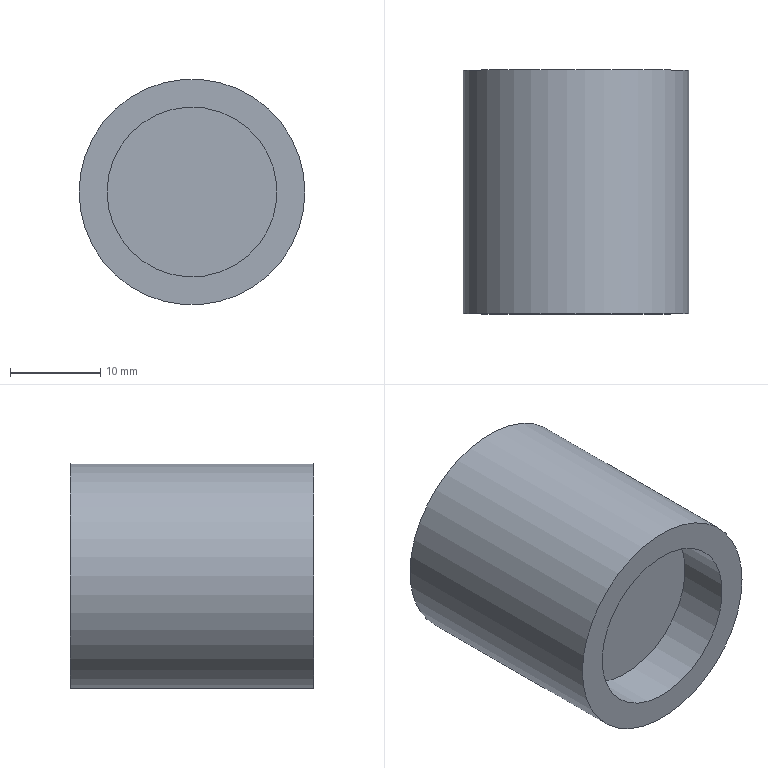Component | NX | SPRING_SEAT | 1 solid | 9 faces | box 25 x 27 x 25 mm | volume 9515 mm3 | plane 5 | cylinder 4 | commonest cylinder face diameters 10 x1 15.5 x1 25 x1 18.8 x1
STEP:
#1=CARTESIAN_POINT('',(0.,0.,0.));
#2=DIRECTION('',(0.,0.,1.));
#3=DIRECTION('',(1.,0.,0.));
#4=AXIS2_PLACEMENT_3D('',#1,#2,#3);
#5=CARTESIAN_POINT('',(38.195,58.009,0.));
#6=VERTEX_POINT('',#5);
#7=CARTESIAN_POINT('',(43.195,58.009,0.));
#8=DIRECTION('',(0.,1.,0.));
#9=DIRECTION('',(-1.,0.,0.));
#10=AXIS2_PLACEMENT_3D('',#7,#8,#9);
#11=CIRCLE('',#10,5.);
#12=CARTESIAN_POINT('',(38.195,58.009,0.));
#13=DIRECTION('',(-0.,-1.,0.));
#14=DIRECTION('',(1.,-0.,0.));
#15=AXIS2_PLACEMENT_3D('',#12,#13,#14);
#16=PLANE('',#15);
#17=CARTESIAN_POINT('',(0.,0.));
#18=CARTESIAN_POINT('',(0.,8.66));
#19=CARTESIAN_POINT('',(7.5,4.33));
#20=CARTESIAN_POINT('',(15.,0.));
#21=CARTESIAN_POINT('',(7.5,-4.33));
#22=CARTESIAN_POINT('',(0.,-8.66));
#23=CARTESIAN_POINT('',(0.,0.));
#24=(BOUNDED_CURVE()B_SPLINE_CURVE(2,(#17,#18,#19,#20,#21,#22,#23),.UNSPECIFIED.,.T.,.F.)B_SPLINE_CURVE_WITH_KNOTS((1,2,2,2,2,1),(-2.094,0.,2.094,4.189,6.283,8.378),.UNSPECIFIED.)CURVE()GEOMETRIC_REPRESENTATION_ITEM()RATIONAL_B_SPLINE_CURVE((1.,0.5,1.,0.5,1.,0.5,1.))REPRESENTATION_ITEM(''));
#25=(GEOMETRIC_REPRESENTATION_CONTEXT(2)PARAMETRIC_REPRESENTATION_CONTEXT()REPRESENTATION_CONTEXT('',''));
#26=DEFINITIONAL_REPRESENTATION('',(#24),#25);
#27=PCURVE('',#16,#26);
#28=CARTESIAN_POINT('',(43.195,78.009,0.));
#29=DIRECTION('',(0.,1.,0.));
#30=DIRECTION('',(-1.,0.,0.));
#31=AXIS2_PLACEMENT_3D('',#28,#29,#30);
#32=CYLINDRICAL_SURFACE('',#31,5.);
#33=CARTESIAN_POINT('',(0.,-20.));
#34=DIRECTION('',(1.,0.));
#35=VECTOR('',#34,1.);
#36=LINE('',#33,#35);
#37=(GEOMETRIC_REPRESENTATION_CONTEXT(2)PARAMETRIC_REPRESENTATION_CONTEXT()REPRESENTATION_CONTEXT('',''));
#38=DEFINITIONAL_REPRESENTATION('',(#36),#37);
#39=PCURVE('',#32,#38);
#40=SURFACE_CURVE('',#11,(#27,#39),.PCURVE_S1.);
#41=EDGE_CURVE('',#6,#6,#40,.T.);
#42=ORIENTED_EDGE('',*,*,#41,.T.);
#43=EDGE_LOOP('',(#42));
#44=FACE_BOUND('',#43,.T.);
#45=ADVANCED_FACE('',(#44),#16,.F.);
#46=ORIENTED_EDGE('',*,*,#41,.T.);
#47=CARTESIAN_POINT('',(38.195,67.809,0.));
#48=VERTEX_POINT('',#47);
#49=CARTESIAN_POINT('',(38.195,58.009,0.));
#50=CARTESIAN_POINT('',(38.195,67.809,0.));
#51=B_SPLINE_CURVE_WITH_KNOTS('',1,(#49,#50),.UNSPECIFIED.,.F.,.F.,(2,2),(-20.,-10.2),.PIECEWISE_BEZIER_KNOTS.);
#52=CARTESIAN_POINT('',(6.283,0.));
#53=DIRECTION('',(0.,1.));
#54=VECTOR('',#53,1.);
#55=LINE('',#52,#54);
#56=(GEOMETRIC_REPRESENTATION_CONTEXT(2)PARAMETRIC_REPRESENTATION_CONTEXT()REPRESENTATION_CONTEXT('',''));
#57=DEFINITIONAL_REPRESENTATION('',(#55),#56);
#58=PCURVE('',#32,#57);
#59=CARTESIAN_POINT('',(0.,0.));
#60=DIRECTION('',(0.,1.));
#61=VECTOR('',#60,1.);
#62=LINE('',#59,#61);
#63=(GEOMETRIC_REPRESENTATION_CONTEXT(2)PARAMETRIC_REPRESENTATION_CONTEXT()REPRESENTATION_CONTEXT('',''));
#64=DEFINITIONAL_REPRESENTATION('',(#62),#63);
#65=PCURVE('',#32,#64);
#66=SEAM_CURVE('',#51,(#58,#65),.PCURVE_S1.);
#67=EDGE_CURVE('',#6,#48,#66,.T.);
#68=ORIENTED_EDGE('',*,*,#67,.T.);
#69=CARTESIAN_POINT('',(43.195,67.809,0.));
#70=DIRECTION('',(0.,1.,0.));
#71=DIRECTION('',(-1.,0.,0.));
#72=AXIS2_PLACEMENT_3D('',#69,#70,#71);
#73=CIRCLE('',#72,5.);
#74=CARTESIAN_POINT('',(0.,-10.2));
#75=DIRECTION('',(1.,0.));
#76=VECTOR('',#75,1.);
#77=LINE('',#74,#76);
#78=(GEOMETRIC_REPRESENTATION_CONTEXT(2)PARAMETRIC_REPRESENTATION_CONTEXT()REPRESENTATION_CONTEXT('',''));
#79=DEFINITIONAL_REPRESENTATION('',(#77),#78);
#80=PCURVE('',#32,#79);
#81=CARTESIAN_POINT('',(35.445,67.809,0.));
#82=DIRECTION('',(-0.,-1.,0.));
#83=DIRECTION('',(1.,-0.,0.));
#84=AXIS2_PLACEMENT_3D('',#81,#82,#83);
#85=PLANE('',#84);
#86=CARTESIAN_POINT('',(2.75,0.));
#87=CARTESIAN_POINT('',(2.75,8.66));
#88=CARTESIAN_POINT('',(10.25,4.33));
#89=CARTESIAN_POINT('',(17.75,0.));
#90=CARTESIAN_POINT('',(10.25,-4.33));
#91=CARTESIAN_POINT('',(2.75,-8.66));
#92=CARTESIAN_POINT('',(2.75,0.));
#93=(BOUNDED_CURVE()B_SPLINE_CURVE(2,(#86,#87,#88,#89,#90,#91,#92),.UNSPECIFIED.,.T.,.F.)B_SPLINE_CURVE_WITH_KNOTS((1,2,2,2,2,1),(-2.094,0.,2.094,4.189,6.283,8.378),.UNSPECIFIED.)CURVE()GEOMETRIC_REPRESENTATION_ITEM()RATIONAL_B_SPLINE_CURVE((1.,0.5,1.,0.5,1.,0.5,1.))REPRESENTATION_ITEM(''));
#94=(GEOMETRIC_REPRESENTATION_CONTEXT(2)PARAMETRIC_REPRESENTATION_CONTEXT()REPRESENTATION_CONTEXT('',''));
#95=DEFINITIONAL_REPRESENTATION('',(#93),#94);
#96=PCURVE('',#85,#95);
#97=SURFACE_CURVE('',#73,(#80,#96),.PCURVE_S1.);
#98=EDGE_CURVE('',#48,#48,#97,.T.);
#99=ORIENTED_EDGE('',*,*,#98,.F.);
#100=ORIENTED_EDGE('',*,*,#67,.F.);
#101=EDGE_LOOP('',(#46,#68,#99,#100));
#102=FACE_BOUND('',#101,.F.);
#103=ADVANCED_FACE('',(#102),#32,.F.);
#104=ORIENTED_EDGE('',*,*,#98,.F.);
#105=EDGE_LOOP('',(#104));
#106=FACE_BOUND('',#105,.T.);
#107=CARTESIAN_POINT('',(35.445,67.809,0.));
#108=VERTEX_POINT('',#107);
#109=CARTESIAN_POINT('',(43.195,67.809,0.));
#110=DIRECTION('',(0.,1.,0.));
#111=DIRECTION('',(-1.,0.,0.));
#112=AXIS2_PLACEMENT_3D('',#109,#110,#111);
#113=CIRCLE('',#112,7.75);
#114=CARTESIAN_POINT('',(0.,0.));
#115=CARTESIAN_POINT('',(0.,13.423));
#116=CARTESIAN_POINT('',(11.625,6.712));
#117=CARTESIAN_POINT('',(23.25,0.));
#118=CARTESIAN_POINT('',(11.625,-6.712));
#119=CARTESIAN_POINT('',(0.,-13.423));
#120=CARTESIAN_POINT('',(0.,0.));
#121=(BOUNDED_CURVE()B_SPLINE_CURVE(2,(#114,#115,#116,#117,#118,#119,#120),.UNSPECIFIED.,.T.,.F.)B_SPLINE_CURVE_WITH_KNOTS((1,2,2,2,2,1),(-2.094,0.,2.094,4.189,6.283,8.378),.UNSPECIFIED.)CURVE()GEOMETRIC_REPRESENTATION_ITEM()RATIONAL_B_SPLINE_CURVE((1.,0.5,1.,0.5,1.,0.5,1.))REPRESENTATION_ITEM(''));
#122=(GEOMETRIC_REPRESENTATION_CONTEXT(2)PARAMETRIC_REPRESENTATION_CONTEXT()REPRESENTATION_CONTEXT('',''));
#123=DEFINITIONAL_REPRESENTATION('',(#121),#122);
#124=PCURVE('',#85,#123);
#125=CARTESIAN_POINT('',(43.195,78.009,0.));
#126=DIRECTION('',(0.,1.,0.));
#127=DIRECTION('',(-1.,0.,0.));
#128=AXIS2_PLACEMENT_3D('',#125,#126,#127);
#129=CYLINDRICAL_SURFACE('',#128,7.75);
#130=CARTESIAN_POINT('',(0.,-10.2));
#131=DIRECTION('',(1.,0.));
#132=VECTOR('',#131,1.);
#133=LINE('',#130,#132);
#134=(GEOMETRIC_REPRESENTATION_CONTEXT(2)PARAMETRIC_REPRESENTATION_CONTEXT()REPRESENTATION_CONTEXT('',''));
#135=DEFINITIONAL_REPRESENTATION('',(#133),#134);
#136=PCURVE('',#129,#135);
#137=SURFACE_CURVE('',#113,(#124,#136),.PCURVE_S1.);
#138=EDGE_CURVE('',#108,#108,#137,.T.);
#139=ORIENTED_EDGE('',*,*,#138,.T.);
#140=EDGE_LOOP('',(#139));
#141=FACE_BOUND('',#140,.T.);
#142=ADVANCED_FACE('',(#106,#141),#85,.F.);
#143=ORIENTED_EDGE('',*,*,#138,.T.);
#144=CARTESIAN_POINT('',(35.445,75.009,0.));
#145=VERTEX_POINT('',#144);
#146=CARTESIAN_POINT('',(35.445,67.809,0.));
#147=CARTESIAN_POINT('',(35.445,75.009,0.));
#148=B_SPLINE_CURVE_WITH_KNOTS('',1,(#146,#147),.UNSPECIFIED.,.F.,.F.,(2,2),(-10.2,-3.),.PIECEWISE_BEZIER_KNOTS.);
#149=CARTESIAN_POINT('',(6.283,0.));
#150=DIRECTION('',(0.,1.));
#151=VECTOR('',#150,1.);
#152=LINE('',#149,#151);
#153=(GEOMETRIC_REPRESENTATION_CONTEXT(2)PARAMETRIC_REPRESENTATION_CONTEXT()REPRESENTATION_CONTEXT('',''));
#154=DEFINITIONAL_REPRESENTATION('',(#152),#153);
#155=PCURVE('',#129,#154);
#156=CARTESIAN_POINT('',(0.,0.));
#157=DIRECTION('',(0.,1.));
#158=VECTOR('',#157,1.);
#159=LINE('',#156,#158);
#160=(GEOMETRIC_REPRESENTATION_CONTEXT(2)PARAMETRIC_REPRESENTATION_CONTEXT()REPRESENTATION_CONTEXT('',''));
#161=DEFINITIONAL_REPRESENTATION('',(#159),#160);
#162=PCURVE('',#129,#161);
#163=SEAM_CURVE('',#148,(#155,#162),.PCURVE_S1.);
#164=EDGE_CURVE('',#108,#145,#163,.T.);
#165=ORIENTED_EDGE('',*,*,#164,.T.);
#166=CARTESIAN_POINT('',(43.195,75.009,0.));
#167=DIRECTION('',(0.,1.,0.));
#168=DIRECTION('',(-1.,0.,0.));
#169=AXIS2_PLACEMENT_3D('',#166,#167,#168);
#170=CIRCLE('',#169,7.75);
#171=CARTESIAN_POINT('',(0.,-3.));
#172=DIRECTION('',(1.,0.));
#173=VECTOR('',#172,1.);
#174=LINE('',#171,#173);
#175=(GEOMETRIC_REPRESENTATION_CONTEXT(2)PARAMETRIC_REPRESENTATION_CONTEXT()REPRESENTATION_CONTEXT('',''));
#176=DEFINITIONAL_REPRESENTATION('',(#174),#175);
#177=PCURVE('',#129,#176);
#178=CARTESIAN_POINT('',(30.695,75.009,0.));
#179=DIRECTION('',(-0.,-1.,0.));
#180=DIRECTION('',(1.,-0.,0.));
#181=AXIS2_PLACEMENT_3D('',#178,#179,#180);
#182=PLANE('',#181);
#183=CARTESIAN_POINT('',(4.75,0.));
#184=CARTESIAN_POINT('',(4.75,13.423));
#185=CARTESIAN_POINT('',(16.375,6.712));
#186=CARTESIAN_POINT('',(28.,0.));
#187=CARTESIAN_POINT('',(16.375,-6.712));
#188=CARTESIAN_POINT('',(4.75,-13.423));
#189=CARTESIAN_POINT('',(4.75,0.));
#190=(BOUNDED_CURVE()B_SPLINE_CURVE(2,(#183,#184,#185,#186,#187,#188,#189),.UNSPECIFIED.,.T.,.F.)B_SPLINE_CURVE_WITH_KNOTS((1,2,2,2,2,1),(-2.094,0.,2.094,4.189,6.283,8.378),.UNSPECIFIED.)CURVE()GEOMETRIC_REPRESENTATION_ITEM()RATIONAL_B_SPLINE_CURVE((1.,0.5,1.,0.5,1.,0.5,1.))REPRESENTATION_ITEM(''));
#191=(GEOMETRIC_REPRESENTATION_CONTEXT(2)PARAMETRIC_REPRESENTATION_CONTEXT()REPRESENTATION_CONTEXT('',''));
#192=DEFINITIONAL_REPRESENTATION('',(#190),#191);
#193=PCURVE('',#182,#192);
#194=SURFACE_CURVE('',#170,(#177,#193),.PCURVE_S1.);
#195=EDGE_CURVE('',#145,#145,#194,.T.);
#196=ORIENTED_EDGE('',*,*,#195,.F.);
#197=ORIENTED_EDGE('',*,*,#164,.F.);
#198=EDGE_LOOP('',(#143,#165,#196,#197));
#199=FACE_BOUND('',#198,.F.);
#200=ADVANCED_FACE('',(#199),#129,.F.);
#201=ORIENTED_EDGE('',*,*,#195,.F.);
#202=EDGE_LOOP('',(#201));
#203=FACE_BOUND('',#202,.T.);
#204=CARTESIAN_POINT('',(30.695,75.009,0.));
#205=VERTEX_POINT('',#204);
#206=CARTESIAN_POINT('',(43.195,75.009,0.));
#207=DIRECTION('',(0.,1.,0.));
#208=DIRECTION('',(-1.,0.,0.));
#209=AXIS2_PLACEMENT_3D('',#206,#207,#208);
#210=CIRCLE('',#209,12.5);
#211=CARTESIAN_POINT('',(0.,0.));
#212=CARTESIAN_POINT('',(0.,21.651));
#213=CARTESIAN_POINT('',(18.75,10.825));
#214=CARTESIAN_POINT('',(37.5,0.));
#215=CARTESIAN_POINT('',(18.75,-10.825));
#216=CARTESIAN_POINT('',(0.,-21.651));
#217=CARTESIAN_POINT('',(0.,0.));
#218=(BOUNDED_CURVE()B_SPLINE_CURVE(2,(#211,#212,#213,#214,#215,#216,#217),.UNSPECIFIED.,.T.,.F.)B_SPLINE_CURVE_WITH_KNOTS((1,2,2,2,2,1),(-2.094,0.,2.094,4.189,6.283,8.378),.UNSPECIFIED.)CURVE()GEOMETRIC_REPRESENTATION_ITEM()RATIONAL_B_SPLINE_CURVE((1.,0.5,1.,0.5,1.,0.5,1.))REPRESENTATION_ITEM(''));
#219=(GEOMETRIC_REPRESENTATION_CONTEXT(2)PARAMETRIC_REPRESENTATION_CONTEXT()REPRESENTATION_CONTEXT('',''));
#220=DEFINITIONAL_REPRESENTATION('',(#218),#219);
#221=PCURVE('',#182,#220);
#222=CARTESIAN_POINT('',(43.195,78.009,0.));
#223=DIRECTION('',(0.,1.,0.));
#224=DIRECTION('',(-1.,0.,0.));
#225=AXIS2_PLACEMENT_3D('',#222,#223,#224);
#226=CYLINDRICAL_SURFACE('',#225,12.5);
#227=CARTESIAN_POINT('',(0.,-3.));
#228=DIRECTION('',(1.,0.));
#229=VECTOR('',#228,1.);
#230=LINE('',#227,#229);
#231=(GEOMETRIC_REPRESENTATION_CONTEXT(2)PARAMETRIC_REPRESENTATION_CONTEXT()REPRESENTATION_CONTEXT('',''));
#232=DEFINITIONAL_REPRESENTATION('',(#230),#231);
#233=PCURVE('',#226,#232);
#234=SURFACE_CURVE('',#210,(#221,#233),.PCURVE_S1.);
#235=EDGE_CURVE('',#205,#205,#234,.T.);
#236=ORIENTED_EDGE('',*,*,#235,.T.);
#237=EDGE_LOOP('',(#236));
#238=FACE_BOUND('',#237,.T.);
#239=ADVANCED_FACE('',(#203,#238),#182,.F.);
#240=ORIENTED_EDGE('',*,*,#235,.F.);
#241=CARTESIAN_POINT('',(30.695,48.009,0.));
#242=VERTEX_POINT('',#241);
#243=CARTESIAN_POINT('',(30.695,48.009,-0.));
#244=CARTESIAN_POINT('',(30.695,75.009,-0.));
#245=B_SPLINE_CURVE_WITH_KNOTS('',1,(#243,#244),.UNSPECIFIED.,.F.,.F.,(2,2),(-30.,-3.),.PIECEWISE_BEZIER_KNOTS.);
#246=CARTESIAN_POINT('',(0.,0.));
#247=DIRECTION('',(0.,1.));
#248=VECTOR('',#247,1.);
#249=LINE('',#246,#248);
#250=(GEOMETRIC_REPRESENTATION_CONTEXT(2)PARAMETRIC_REPRESENTATION_CONTEXT()REPRESENTATION_CONTEXT('',''));
#251=DEFINITIONAL_REPRESENTATION('',(#249),#250);
#252=PCURVE('',#226,#251);
#253=CARTESIAN_POINT('',(6.283,0.));
#254=DIRECTION('',(0.,1.));
#255=VECTOR('',#254,1.);
#256=LINE('',#253,#255);
#257=(GEOMETRIC_REPRESENTATION_CONTEXT(2)PARAMETRIC_REPRESENTATION_CONTEXT()REPRESENTATION_CONTEXT('',''));
#258=DEFINITIONAL_REPRESENTATION('',(#256),#257);
#259=PCURVE('',#226,#258);
#260=SEAM_CURVE('',#245,(#252,#259),.PCURVE_S1.);
#261=EDGE_CURVE('',#242,#205,#260,.T.);
#262=ORIENTED_EDGE('',*,*,#261,.F.);
#263=CARTESIAN_POINT('',(43.195,48.009,0.));
#264=DIRECTION('',(0.,1.,0.));
#265=DIRECTION('',(-1.,0.,0.));
#266=AXIS2_PLACEMENT_3D('',#263,#264,#265);
#267=CIRCLE('',#266,12.5);
#268=CARTESIAN_POINT('',(0.,-30.));
#269=DIRECTION('',(1.,0.));
#270=VECTOR('',#269,1.);
#271=LINE('',#268,#270);
#272=(GEOMETRIC_REPRESENTATION_CONTEXT(2)PARAMETRIC_REPRESENTATION_CONTEXT()REPRESENTATION_CONTEXT('',''));
#273=DEFINITIONAL_REPRESENTATION('',(#271),#272);
#274=PCURVE('',#226,#273);
#275=CARTESIAN_POINT('',(33.795,48.009,0.));
#276=DIRECTION('',(0.,1.,0.));
#277=DIRECTION('',(-1.,0.,0.));
#278=AXIS2_PLACEMENT_3D('',#275,#276,#277);
#279=PLANE('',#278);
#280=CARTESIAN_POINT('',(-9.4,0.));
#281=DIRECTION('',(1.,0.));
#282=AXIS2_PLACEMENT_2D('',#280,#281);
#283=CIRCLE('',#282,12.5);
#284=(GEOMETRIC_REPRESENTATION_CONTEXT(2)PARAMETRIC_REPRESENTATION_CONTEXT()REPRESENTATION_CONTEXT('',''));
#285=DEFINITIONAL_REPRESENTATION('',(#283),#284);
#286=PCURVE('',#279,#285);
#287=SURFACE_CURVE('',#267,(#274,#286),.PCURVE_S1.);
#288=EDGE_CURVE('',#242,#242,#287,.T.);
#289=ORIENTED_EDGE('',*,*,#288,.T.);
#290=ORIENTED_EDGE('',*,*,#261,.T.);
#291=EDGE_LOOP('',(#240,#262,#289,#290));
#292=FACE_BOUND('',#291,.T.);
#293=ADVANCED_FACE('',(#292),#226,.T.);
#294=ORIENTED_EDGE('',*,*,#288,.F.);
#295=EDGE_LOOP('',(#294));
#296=FACE_BOUND('',#295,.T.);
#297=CARTESIAN_POINT('',(33.795,48.009,0.));
#298=VERTEX_POINT('',#297);
#299=CARTESIAN_POINT('',(43.195,48.009,0.));
#300=DIRECTION('',(0.,1.,0.));
#301=DIRECTION('',(-1.,0.,0.));
#302=AXIS2_PLACEMENT_3D('',#299,#300,#301);
#303=CIRCLE('',#302,9.4);
#304=CARTESIAN_POINT('',(-9.4,0.));
#305=DIRECTION('',(1.,0.));
#306=AXIS2_PLACEMENT_2D('',#304,#305);
#307=CIRCLE('',#306,9.4);
#308=(GEOMETRIC_REPRESENTATION_CONTEXT(2)PARAMETRIC_REPRESENTATION_CONTEXT()REPRESENTATION_CONTEXT('',''));
#309=DEFINITIONAL_REPRESENTATION('',(#307),#308);
#310=PCURVE('',#279,#309);
#311=CARTESIAN_POINT('',(43.195,78.009,0.));
#312=DIRECTION('',(0.,1.,0.));
#313=DIRECTION('',(-1.,0.,0.));
#314=AXIS2_PLACEMENT_3D('',#311,#312,#313);
#315=CYLINDRICAL_SURFACE('',#314,9.4);
#316=CARTESIAN_POINT('',(0.,-30.));
#317=DIRECTION('',(1.,0.));
#318=VECTOR('',#317,1.);
#319=LINE('',#316,#318);
#320=(GEOMETRIC_REPRESENTATION_CONTEXT(2)PARAMETRIC_REPRESENTATION_CONTEXT()REPRESENTATION_CONTEXT('',''));
#321=DEFINITIONAL_REPRESENTATION('',(#319),#320);
#322=PCURVE('',#315,#321);
#323=SURFACE_CURVE('',#303,(#310,#322),.PCURVE_S1.);
#324=EDGE_CURVE('',#298,#298,#323,.T.);
#325=ORIENTED_EDGE('',*,*,#324,.T.);
#326=EDGE_LOOP('',(#325));
#327=FACE_BOUND('',#326,.T.);
#328=ADVANCED_FACE('',(#296,#327),#279,.F.);
#329=ORIENTED_EDGE('',*,*,#324,.T.);
#330=CARTESIAN_POINT('',(33.795,53.809,0.));
#331=VERTEX_POINT('',#330);
#332=CARTESIAN_POINT('',(33.795,48.009,0.));
#333=CARTESIAN_POINT('',(33.795,53.809,0.));
#334=B_SPLINE_CURVE_WITH_KNOTS('',1,(#332,#333),.UNSPECIFIED.,.F.,.F.,(2,2),(-30.,-24.2),.PIECEWISE_BEZIER_KNOTS.);
#335=CARTESIAN_POINT('',(6.283,0.));
#336=DIRECTION('',(0.,1.));
#337=VECTOR('',#336,1.);
#338=LINE('',#335,#337);
#339=(GEOMETRIC_REPRESENTATION_CONTEXT(2)PARAMETRIC_REPRESENTATION_CONTEXT()REPRESENTATION_CONTEXT('',''));
#340=DEFINITIONAL_REPRESENTATION('',(#338),#339);
#341=PCURVE('',#315,#340);
#342=CARTESIAN_POINT('',(0.,0.));
#343=DIRECTION('',(0.,1.));
#344=VECTOR('',#343,1.);
#345=LINE('',#342,#344);
#346=(GEOMETRIC_REPRESENTATION_CONTEXT(2)PARAMETRIC_REPRESENTATION_CONTEXT()REPRESENTATION_CONTEXT('',''));
#347=DEFINITIONAL_REPRESENTATION('',(#345),#346);
#348=PCURVE('',#315,#347);
#349=SEAM_CURVE('',#334,(#341,#348),.PCURVE_S1.);
#350=EDGE_CURVE('',#298,#331,#349,.T.);
#351=ORIENTED_EDGE('',*,*,#350,.T.);
#352=CARTESIAN_POINT('',(43.195,53.809,0.));
#353=DIRECTION('',(0.,1.,0.));
#354=DIRECTION('',(-1.,0.,0.));
#355=AXIS2_PLACEMENT_3D('',#352,#353,#354);
#356=CIRCLE('',#355,9.4);
#357=CARTESIAN_POINT('',(0.,-24.2));
#358=DIRECTION('',(1.,0.));
#359=VECTOR('',#358,1.);
#360=LINE('',#357,#359);
#361=(GEOMETRIC_REPRESENTATION_CONTEXT(2)PARAMETRIC_REPRESENTATION_CONTEXT()REPRESENTATION_CONTEXT('',''));
#362=DEFINITIONAL_REPRESENTATION('',(#360),#361);
#363=PCURVE('',#315,#362);
#364=CARTESIAN_POINT('',(43.195,53.809,0.));
#365=DIRECTION('',(0.,1.,0.));
#366=DIRECTION('',(-1.,0.,0.));
#367=AXIS2_PLACEMENT_3D('',#364,#365,#366);
#368=PLANE('',#367);
#369=CARTESIAN_POINT('',(0.,0.));
#370=DIRECTION('',(1.,0.));
#371=AXIS2_PLACEMENT_2D('',#369,#370);
#372=CIRCLE('',#371,9.4);
#373=(GEOMETRIC_REPRESENTATION_CONTEXT(2)PARAMETRIC_REPRESENTATION_CONTEXT()REPRESENTATION_CONTEXT('',''));
#374=DEFINITIONAL_REPRESENTATION('',(#372),#373);
#375=PCURVE('',#368,#374);
#376=SURFACE_CURVE('',#356,(#363,#375),.PCURVE_S1.);
#377=EDGE_CURVE('',#331,#331,#376,.T.);
#378=ORIENTED_EDGE('',*,*,#377,.F.);
#379=ORIENTED_EDGE('',*,*,#350,.F.);
#380=EDGE_LOOP('',(#329,#351,#378,#379));
#381=FACE_BOUND('',#380,.F.);
#382=ADVANCED_FACE('',(#381),#315,.F.);
#383=ORIENTED_EDGE('',*,*,#377,.F.);
#384=EDGE_LOOP('',(#383));
#385=FACE_BOUND('',#384,.T.);
#386=ADVANCED_FACE('',(#385),#368,.F.);
#387=CLOSED_SHELL('',(#45,#103,#142,#200,#239,#293,#328,#382,#386));
#388=MANIFOLD_SOLID_BREP('',#387);
#389=(LENGTH_UNIT()NAMED_UNIT(*)SI_UNIT(.MILLI.,.METRE.));
#390=UNCERTAINTY_MEASURE_WITH_UNIT(LENGTH_MEASURE(0.00001),#389,'','');
#391=(NAMED_UNIT(*)PLANE_ANGLE_UNIT()SI_UNIT($,.RADIAN.));
#392=(NAMED_UNIT(*)SI_UNIT($,.STERADIAN.)SOLID_ANGLE_UNIT());
#393=(GEOMETRIC_REPRESENTATION_CONTEXT(3)GLOBAL_UNCERTAINTY_ASSIGNED_CONTEXT((#390))GLOBAL_UNIT_ASSIGNED_CONTEXT((#389,#391,#392))REPRESENTATION_CONTEXT('',''));
#394=ADVANCED_BREP_SHAPE_REPRESENTATION('',(#4,#388),#393);